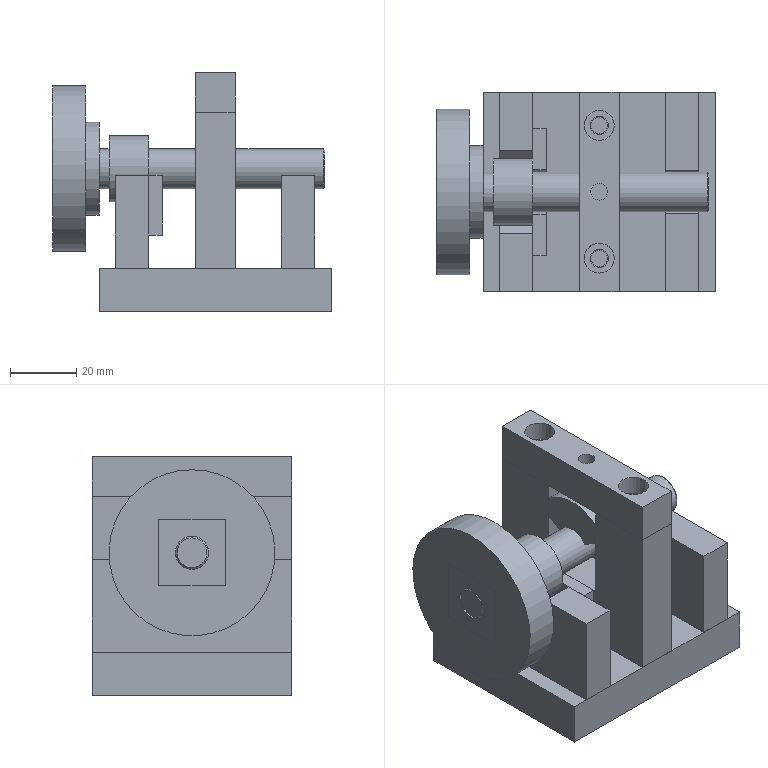Assembly | NX | mm | 11 component files | 11 solids | 155 faces | box 84 x 60 x 72 mm | volume 146807 mm3 | plane 96 | cylinder 57 | cone 2 | commonest cylinder face diameters 5 x21 9 x9 5.5 x8 6 x4 12 x3 10 x3 4 x2 4.5 x2
Bill of materials:
unnamed part 1 | 1 |  | Solid stepped cylindrical shaft/pin: a long plain cylindrical section, a short larger-diameter collar, a short intermediate step, a narrow groove, and a smaller-diameter end spigot.
unnamed part 2 | 1 |  | Rectangular bar with three round holes in a line along its length, perpendicular to the top face; the two end holes look larger than the center hole.
unnamed part 3 | 1 |  | U-shaped block (clevis-like form): a rectangular base with two upright prongs on either side of a central rectangular slot, and a small hole in the top face of each prong.
unnamed part 4 | 1 |  | Flat circular ring/washer-like disc with a central round through hole.
unnamed part 5 | 1 |  | Rectangular block with a single large round through hole running through its thickness, perpendicular to the largest face.
unnamed part 6 | 1 |  | Flat circular disc with a central square through hole.
unnamed part 7 | 1 |  | Rectangular plate with a semicircular cutout centered on one long edge and two round through holes, one on each side of the cutout.
unnamed part 8 | 1 |  | Rectangular block with a deep symmetric V-groove along its top edge, and two small round through holes on either side of the groove.
unnamed part 9 | 1 |  | Rectangular block with a shallow symmetric V-notch along its top edge; no holes are visible.
unnamed part 10 | 1 |  | Thick square-to-rectangular plate with 15 round through holes in three columns of five, mixing larger and smaller hole sizes.
unnamed part 11 | 1 |  | Saddle-shaped block: a convex curved top, a concave arc-shaped cutout on the bottom, flat ends and flat sides, and one round hole entering the curved top face.
Mates:
1. fix | base 1 component
2. concentric | rear_bracket 1 arc | base 1 edge
3. parallel | rear_bracket 1 face | base 1 face
4. concentric | base 1 edge | front_bracket 1 arc
5. parallel | front_bracket 1 face | base 1 face
6. concentric | baffle_plate 1 arc | front_bracket 1 edge
7. parallel | baffle_plate 1 face | front_bracket 1 face
8. concentric | base 1 edge | U_plate 1 arc
9. parallel | U_plate 1 face | front_bracket 1 face
10. concentric | U_plate 1 arc | cover_plate 1 arc
11. parallel | cover_plate 1 face | U_plate 1 face
12. touch align | spindle 1 face | baffle_plate 1 face
13. touch align | spindle 1 face | baffle_plate 1 face
14. concentric | spindle 1 edge | support_ring 1 arc
15. concentric | support_ring 1 edge | bushing 1 edge
16. touch align | faceplate 1 face | bushing 1 face
17. touch align | faceplate 1 face | bushing 1 face
18. touch align | faceplate 1 face | bushing 1 face
19. touch align | bearing_bush 1 face | cover_plate 1 face
20. touch align | spindle 1 face | bearing_bush 1 face